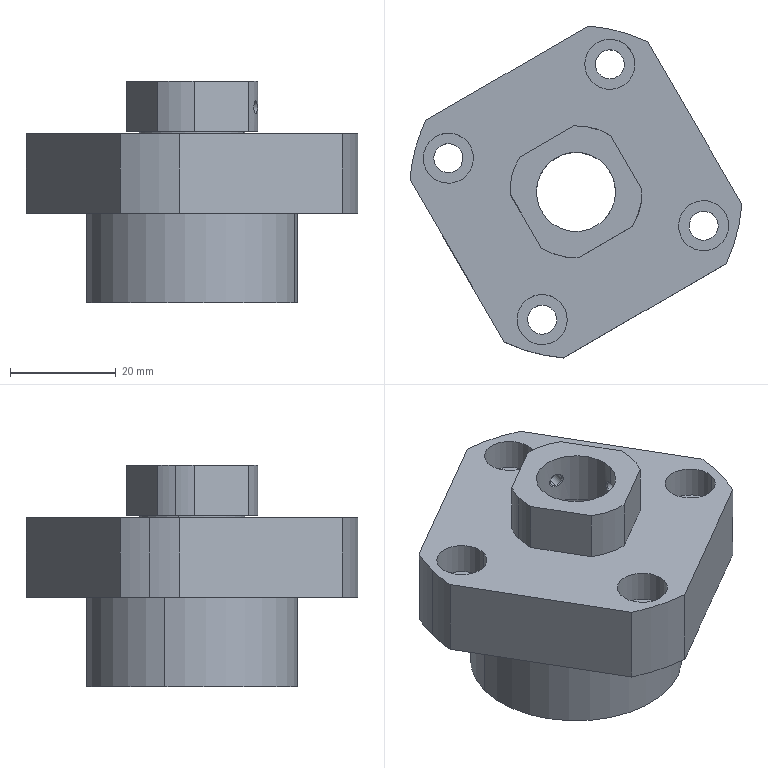Component | SolidWorks | FK15BallScrewSupportUnit(FixedSide)0-1 | 1 solid | 108 faces | volume 50504 mm3 | cylinder 58 | plane 24 | spline 18 | cone 6 | torus 2 | commonest cylinder face diameters 9.5 x8 5.5 x8 15 x6 32 x6 63 x5 25 x5 2.459 x4 26.1 x4